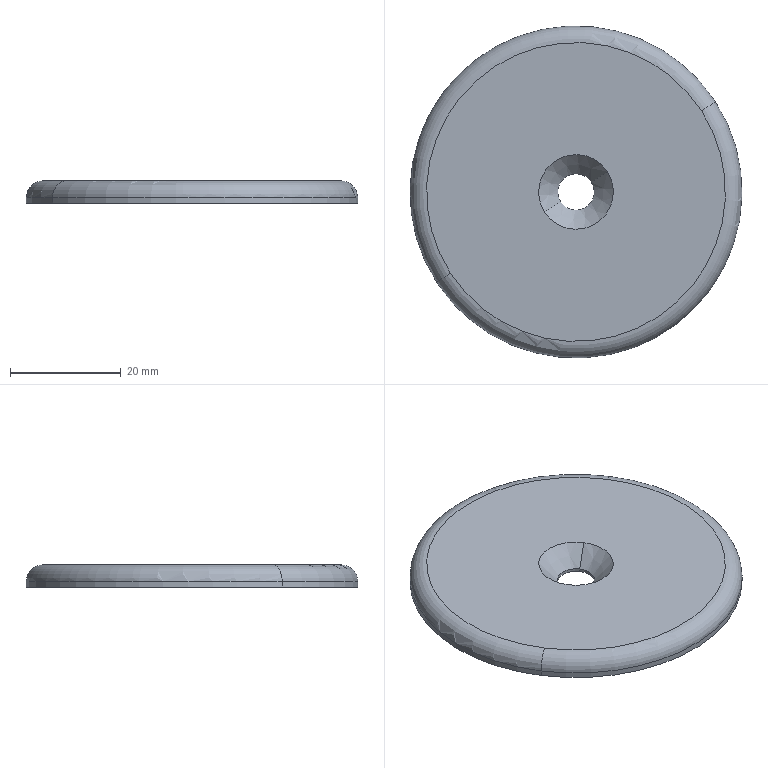Component | SolidWorks | JYTBJ-HeaderPlateAxisBarrelCover-1 | 1 solid | 10 faces | box 60 x 60 x 4 mm | volume 10651 mm3 | cylinder 4 | torus 2 | cone 2 | plane 2 | commonest cylinder face diameters 6.6 x2 60 x2
build123d program:
from build123d import *

# Parameters (mm, degrees)
SKETCH1_R           = 30
BOSS_EXTRUDE1_DEPTH = 2
FILLET1_R           = 3


with BuildPart() as part:
    # Sketch1 → Boss-Extrude1 (new, symmetric)
    with BuildSketch(Plane.XY):
        Circle(SKETCH1_R)
    extrude(amount=BOSS_EXTRUDE1_DEPTH, both=True)

    # Sketch2 → Hole Size according to Hexagon Socket Ra (revolve, cut)
    with BuildSketch(Plane(origin=(0, 0, 2), x_dir=(0, -1, 0), z_dir=(1, 0, 0))):
        Polygon((0, 0), (0, 4), (3.3, 4), (3.3, 3.45), (6.75, 0), align=None)
    revolve(axis=Axis((0, 0, 8.35), (0, 0, -1)), mode=Mode.SUBTRACT)

    # Fillet1
    fillet1_edges = [part.edges().sort_by_distance(p)[0] for p in [
        (-30, 0, 2),
    ]]
    fillet(fillet1_edges, radius=FILLET1_R)


solid = part.part

# Placed as in the assembly
solid = solid.moved(Location((3.373, 96.878, 260.5), (0, 0, 0)))
STEP:
#1=COLOUR_RGB('',0.7922,0.8196,0.9333);
#2=FILL_AREA_STYLE_COLOUR('',#1);
#3=FILL_AREA_STYLE('',(#2));
#4=SURFACE_STYLE_FILL_AREA(#3);
#5=SURFACE_SIDE_STYLE('',(#4));
#6=SURFACE_STYLE_USAGE(.BOTH.,#5);
#7=PRESENTATION_STYLE_ASSIGNMENT((#6));
#8=CARTESIAN_POINT('',(-0.8589,3.173,10.217));
#9=VERTEX_POINT('',#8);
#10=CARTESIAN_POINT('',(1.124,4.456,10.217));
#11=VERTEX_POINT('',#10);
#12=CARTESIAN_POINT('',(0.1328,3.814,10.217));
#13=DIRECTION('',(0.,0.,-1.));
#14=DIRECTION('',(0.8396,0.5432,0.));
#15=AXIS2_PLACEMENT_3D('',#12,#13,#14);
#16=CIRCLE('',#15,1.181);
#17=EDGE_CURVE('',#9,#11,#16,.T.);
#18=ORIENTED_EDGE('',*,*,#17,.F.);
#19=CARTESIAN_POINT('',(-0.7597,3.237,10.335));
#20=VERTEX_POINT('',#19);
#21=CARTESIAN_POINT('',(-0.7597,3.237,10.217));
#22=DIRECTION('',(-0.5432,0.8396,0.));
#23=DIRECTION('',(-0.8396,-0.5432,0.));
#24=AXIS2_PLACEMENT_3D('',#21,#22,#23);
#25=CIRCLE('',#24,0.1181);
#26=EDGE_CURVE('',#9,#20,#25,.T.);
#27=ORIENTED_EDGE('',*,*,#26,.T.);
#28=CARTESIAN_POINT('',(1.025,4.391,10.335));
#29=VERTEX_POINT('',#28);
#30=CARTESIAN_POINT('',(0.1328,3.814,10.335));
#31=DIRECTION('',(0.,0.,1.));
#32=DIRECTION('',(0.8396,0.5432,0.));
#33=AXIS2_PLACEMENT_3D('',#30,#31,#32);
#34=CIRCLE('',#33,1.063);
#35=EDGE_CURVE('',#29,#20,#34,.T.);
#36=ORIENTED_EDGE('',*,*,#35,.F.);
#37=CARTESIAN_POINT('',(1.025,4.391,10.217));
#38=DIRECTION('',(0.5432,-0.8396,0.));
#39=DIRECTION('',(0.8396,0.5432,0.));
#40=AXIS2_PLACEMENT_3D('',#37,#38,#39);
#41=CIRCLE('',#40,0.1181);
#42=EDGE_CURVE('',#11,#29,#41,.T.);
#43=ORIENTED_EDGE('',*,*,#42,.F.);
#44=EDGE_LOOP('',(#18,#27,#36,#43));
#45=FACE_OUTER_BOUND('',#44,.T.);
#46=CARTESIAN_POINT('',(0.1328,3.814,10.217));
#47=DIRECTION('',(0.,0.,1.));
#48=DIRECTION('',(0.8396,0.5432,0.));
#49=AXIS2_PLACEMENT_3D('',#46,#47,#48);
#50=TOROIDAL_SURFACE('',#49,1.063,0.1181);
#51=ADVANCED_FACE('',(#45),#50,.T.);
#52=CARTESIAN_POINT('',(0.02373,3.744,10.199));
#53=VERTEX_POINT('',#52);
#54=CARTESIAN_POINT('',(0.2419,3.885,10.199));
#55=VERTEX_POINT('',#54);
#56=CARTESIAN_POINT('',(0.1328,3.814,10.199));
#57=DIRECTION('',(0.,0.,1.));
#58=DIRECTION('',(0.8396,0.5432,0.));
#59=AXIS2_PLACEMENT_3D('',#56,#57,#58);
#60=CIRCLE('',#59,0.1299);
#61=EDGE_CURVE('',#53,#55,#60,.T.);
#62=ORIENTED_EDGE('',*,*,#61,.F.);
#63=CARTESIAN_POINT('',(-0.09032,3.67,10.335));
#64=VERTEX_POINT('',#63);
#65=CARTESIAN_POINT('',(-0.09032,3.67,10.335));
#66=DIRECTION('',(-0.5937,-0.3841,0.7071));
#67=VECTOR('',#66,39.37);
#68=LINE('',#65,#67);
#69=EDGE_CURVE('',#53,#64,#68,.T.);
#70=ORIENTED_EDGE('',*,*,#69,.T.);
#71=CARTESIAN_POINT('',(0.3559,3.958,10.335));
#72=VERTEX_POINT('',#71);
#73=CARTESIAN_POINT('',(0.1328,3.814,10.335));
#74=DIRECTION('',(0.,0.,1.));
#75=DIRECTION('',(0.8396,0.5432,0.));
#76=AXIS2_PLACEMENT_3D('',#73,#74,#75);
#77=CIRCLE('',#76,0.2657);
#78=EDGE_CURVE('',#64,#72,#77,.T.);
#79=ORIENTED_EDGE('',*,*,#78,.T.);
#80=CARTESIAN_POINT('',(0.3559,3.958,10.335));
#81=DIRECTION('',(0.5937,0.3841,0.7071));
#82=VECTOR('',#81,39.37);
#83=LINE('',#80,#82);
#84=EDGE_CURVE('',#55,#72,#83,.T.);
#85=ORIENTED_EDGE('',*,*,#84,.F.);
#86=EDGE_LOOP('',(#62,#70,#79,#85));
#87=FACE_OUTER_BOUND('',#86,.T.);
#88=CARTESIAN_POINT('',(0.1328,3.814,10.335));
#89=DIRECTION('',(0.,0.,1.));
#90=DIRECTION('',(0.8396,0.5432,0.));
#91=AXIS2_PLACEMENT_3D('',#88,#89,#90);
#92=CONICAL_SURFACE('',#91,0.2657,0.7854);
#93=ADVANCED_FACE('',(#87),#92,.F.);
#94=CARTESIAN_POINT('',(0.02373,3.744,10.177));
#95=VERTEX_POINT('',#94);
#96=CARTESIAN_POINT('',(0.2419,3.885,10.177));
#97=VERTEX_POINT('',#96);
#98=CARTESIAN_POINT('',(0.1328,3.814,10.177));
#99=DIRECTION('',(0.,0.,1.));
#100=DIRECTION('',(0.8396,0.5432,0.));
#101=AXIS2_PLACEMENT_3D('',#98,#99,#100);
#102=CIRCLE('',#101,0.1299);
#103=EDGE_CURVE('',#95,#97,#102,.T.);
#104=ORIENTED_EDGE('',*,*,#103,.F.);
#105=CARTESIAN_POINT('',(0.02373,3.744,10.335));
#106=DIRECTION('',(0.,0.,1.));
#107=VECTOR('',#106,39.37);
#108=LINE('',#105,#107);
#109=EDGE_CURVE('',#95,#53,#108,.T.);
#110=ORIENTED_EDGE('',*,*,#109,.T.);
#111=ORIENTED_EDGE('',*,*,#61,.T.);
#112=CARTESIAN_POINT('',(0.2419,3.885,10.335));
#113=DIRECTION('',(0.,0.,1.));
#114=VECTOR('',#113,39.37);
#115=LINE('',#112,#114);
#116=EDGE_CURVE('',#97,#55,#115,.T.);
#117=ORIENTED_EDGE('',*,*,#116,.F.);
#118=EDGE_LOOP('',(#104,#110,#111,#117));
#119=FACE_OUTER_BOUND('',#118,.T.);
#120=CARTESIAN_POINT('',(0.1328,3.814,10.335));
#121=DIRECTION('',(0.,0.,1.));
#122=DIRECTION('',(0.8396,0.5432,0.));
#123=AXIS2_PLACEMENT_3D('',#120,#121,#122);
#124=CYLINDRICAL_SURFACE('',#123,0.1299);
#125=ADVANCED_FACE('',(#119),#124,.F.);
#126=ORIENTED_EDGE('',*,*,#17,.T.);
#127=CARTESIAN_POINT('',(1.124,4.456,10.177));
#128=VERTEX_POINT('',#127);
#129=CARTESIAN_POINT('',(1.124,4.456,10.335));
#130=DIRECTION('',(0.,0.,-1.));
#131=VECTOR('',#130,39.37);
#132=LINE('',#129,#131);
#133=EDGE_CURVE('',#11,#128,#132,.T.);
#134=ORIENTED_EDGE('',*,*,#133,.T.);
#135=CARTESIAN_POINT('',(-0.8589,3.173,10.177));
#136=VERTEX_POINT('',#135);
#137=CARTESIAN_POINT('',(0.1328,3.814,10.177));
#138=DIRECTION('',(0.,0.,1.));
#139=DIRECTION('',(0.8396,0.5432,0.));
#140=AXIS2_PLACEMENT_3D('',#137,#138,#139);
#141=CIRCLE('',#140,1.181);
#142=EDGE_CURVE('',#128,#136,#141,.T.);
#143=ORIENTED_EDGE('',*,*,#142,.T.);
#144=CARTESIAN_POINT('',(-0.8589,3.173,10.335));
#145=DIRECTION('',(0.,0.,-1.));
#146=VECTOR('',#145,39.37);
#147=LINE('',#144,#146);
#148=EDGE_CURVE('',#9,#136,#147,.T.);
#149=ORIENTED_EDGE('',*,*,#148,.F.);
#150=EDGE_LOOP('',(#126,#134,#143,#149));
#151=FACE_OUTER_BOUND('',#150,.T.);
#152=CARTESIAN_POINT('',(0.1328,3.814,10.335));
#153=DIRECTION('',(0.,0.,-1.));
#154=DIRECTION('',(-0.8396,-0.5432,0.));
#155=AXIS2_PLACEMENT_3D('',#152,#153,#154);
#156=CYLINDRICAL_SURFACE('',#155,1.181);
#157=ADVANCED_FACE('',(#151),#156,.T.);
#158=ORIENTED_EDGE('',*,*,#133,.F.);
#159=CARTESIAN_POINT('',(0.1328,3.814,10.217));
#160=DIRECTION('',(0.,0.,-1.));
#161=DIRECTION('',(0.8396,0.5432,0.));
#162=AXIS2_PLACEMENT_3D('',#159,#160,#161);
#163=CIRCLE('',#162,1.181);
#164=EDGE_CURVE('',#11,#9,#163,.T.);
#165=ORIENTED_EDGE('',*,*,#164,.T.);
#166=ORIENTED_EDGE('',*,*,#148,.T.);
#167=CARTESIAN_POINT('',(0.1328,3.814,10.177));
#168=DIRECTION('',(0.,0.,1.));
#169=DIRECTION('',(0.8396,0.5432,0.));
#170=AXIS2_PLACEMENT_3D('',#167,#168,#169);
#171=CIRCLE('',#170,1.181);
#172=EDGE_CURVE('',#136,#128,#171,.T.);
#173=ORIENTED_EDGE('',*,*,#172,.T.);
#174=EDGE_LOOP('',(#158,#165,#166,#173));
#175=FACE_OUTER_BOUND('',#174,.T.);
#176=CARTESIAN_POINT('',(0.1328,3.814,10.335));
#177=DIRECTION('',(0.,0.,-1.));
#178=DIRECTION('',(-0.8396,-0.5432,0.));
#179=AXIS2_PLACEMENT_3D('',#176,#177,#178);
#180=CYLINDRICAL_SURFACE('',#179,1.181);
#181=ADVANCED_FACE('',(#175),#180,.T.);
#182=ORIENTED_EDGE('',*,*,#35,.T.);
#183=CARTESIAN_POINT('',(0.1328,3.814,10.335));
#184=DIRECTION('',(0.,0.,1.));
#185=DIRECTION('',(0.8396,0.5432,0.));
#186=AXIS2_PLACEMENT_3D('',#183,#184,#185);
#187=CIRCLE('',#186,1.063);
#188=EDGE_CURVE('',#20,#29,#187,.T.);
#189=ORIENTED_EDGE('',*,*,#188,.T.);
#190=EDGE_LOOP('',(#182,#189));
#191=FACE_OUTER_BOUND('',#190,.T.);
#192=CARTESIAN_POINT('',(0.1328,3.814,10.335));
#193=DIRECTION('',(0.,0.,1.));
#194=DIRECTION('',(0.8396,0.5432,0.));
#195=AXIS2_PLACEMENT_3D('',#192,#193,#194);
#196=CIRCLE('',#195,0.2657);
#197=EDGE_CURVE('',#72,#64,#196,.T.);
#198=ORIENTED_EDGE('',*,*,#197,.F.);
#199=ORIENTED_EDGE('',*,*,#78,.F.);
#200=EDGE_LOOP('',(#198,#199));
#201=FACE_BOUND('',#200,.T.);
#202=CARTESIAN_POINT('',(0.1328,3.814,10.335));
#203=DIRECTION('',(0.,0.,1.));
#204=DIRECTION('',(0.8396,0.5432,0.));
#205=AXIS2_PLACEMENT_3D('',#202,#203,#204);
#206=PLANE('',#205);
#207=ADVANCED_FACE('',(#191,#201),#206,.T.);
#208=CARTESIAN_POINT('',(0.1328,3.814,10.177));
#209=DIRECTION('',(0.,0.,1.));
#210=DIRECTION('',(0.8396,0.5432,0.));
#211=AXIS2_PLACEMENT_3D('',#208,#209,#210);
#212=CIRCLE('',#211,0.1299);
#213=EDGE_CURVE('',#97,#95,#212,.T.);
#214=ORIENTED_EDGE('',*,*,#213,.T.);
#215=ORIENTED_EDGE('',*,*,#103,.T.);
#216=EDGE_LOOP('',(#214,#215));
#217=FACE_BOUND('',#216,.T.);
#218=ORIENTED_EDGE('',*,*,#172,.F.);
#219=ORIENTED_EDGE('',*,*,#142,.F.);
#220=EDGE_LOOP('',(#218,#219));
#221=FACE_OUTER_BOUND('',#220,.T.);
#222=CARTESIAN_POINT('',(0.1328,3.814,10.177));
#223=DIRECTION('',(0.,0.,1.));
#224=DIRECTION('',(0.8396,0.5432,0.));
#225=AXIS2_PLACEMENT_3D('',#222,#223,#224);
#226=PLANE('',#225);
#227=ADVANCED_FACE('',(#217,#221),#226,.F.);
#228=ORIENTED_EDGE('',*,*,#109,.F.);
#229=ORIENTED_EDGE('',*,*,#213,.F.);
#230=ORIENTED_EDGE('',*,*,#116,.T.);
#231=CARTESIAN_POINT('',(0.1328,3.814,10.199));
#232=DIRECTION('',(0.,0.,1.));
#233=DIRECTION('',(0.8396,0.5432,0.));
#234=AXIS2_PLACEMENT_3D('',#231,#232,#233);
#235=CIRCLE('',#234,0.1299);
#236=EDGE_CURVE('',#55,#53,#235,.T.);
#237=ORIENTED_EDGE('',*,*,#236,.T.);
#238=EDGE_LOOP('',(#228,#229,#230,#237));
#239=FACE_OUTER_BOUND('',#238,.T.);
#240=CARTESIAN_POINT('',(0.1328,3.814,10.335));
#241=DIRECTION('',(0.,0.,1.));
#242=DIRECTION('',(0.8396,0.5432,0.));
#243=AXIS2_PLACEMENT_3D('',#240,#241,#242);
#244=CYLINDRICAL_SURFACE('',#243,0.1299);
#245=ADVANCED_FACE('',(#239),#244,.F.);
#246=ORIENTED_EDGE('',*,*,#69,.F.);
#247=ORIENTED_EDGE('',*,*,#236,.F.);
#248=ORIENTED_EDGE('',*,*,#84,.T.);
#249=ORIENTED_EDGE('',*,*,#197,.T.);
#250=EDGE_LOOP('',(#246,#247,#248,#249));
#251=FACE_OUTER_BOUND('',#250,.T.);
#252=CARTESIAN_POINT('',(0.1328,3.814,10.335));
#253=DIRECTION('',(0.,0.,1.));
#254=DIRECTION('',(0.8396,0.5432,0.));
#255=AXIS2_PLACEMENT_3D('',#252,#253,#254);
#256=CONICAL_SURFACE('',#255,0.2657,0.7854);
#257=ADVANCED_FACE('',(#251),#256,.F.);
#258=ORIENTED_EDGE('',*,*,#26,.F.);
#259=ORIENTED_EDGE('',*,*,#164,.F.);
#260=ORIENTED_EDGE('',*,*,#42,.T.);
#261=ORIENTED_EDGE('',*,*,#188,.F.);
#262=EDGE_LOOP('',(#258,#259,#260,#261));
#263=FACE_OUTER_BOUND('',#262,.T.);
#264=CARTESIAN_POINT('',(0.1328,3.814,10.217));
#265=DIRECTION('',(0.,0.,1.));
#266=DIRECTION('',(0.8396,0.5432,0.));
#267=AXIS2_PLACEMENT_3D('',#264,#265,#266);
#268=TOROIDAL_SURFACE('',#267,1.063,0.1181);
#269=ADVANCED_FACE('',(#263),#268,.T.);
#270=CLOSED_SHELL('',(#51,#93,#125,#157,#181,#207,#227,#245,#257,#269));
#271=MANIFOLD_SOLID_BREP('',#270);
#272=STYLED_ITEM('',(#7),#271);
#273=PRESENTATION_LAYER_ASSIGNMENT('','',(#272));
#274=CARTESIAN_POINT('',(0.,0.,0.));
#275=DIRECTION('',(0.,0.,1.));
#276=DIRECTION('',(1.,0.,0.));
#277=AXIS2_PLACEMENT_3D('',#274,#275,#276);
#278=(LENGTH_UNIT()NAMED_UNIT(*)SI_UNIT($,.METRE.));
#279=LENGTH_MEASURE_WITH_UNIT(LENGTH_MEASURE(0.0254),#278);
#280=DIMENSIONAL_EXPONENTS(1.,0.,0.,0.,0.,0.,0.);
#281=(CONVERSION_BASED_UNIT('',#279)LENGTH_UNIT()NAMED_UNIT(#280));
#282=UNCERTAINTY_MEASURE_WITH_UNIT(LENGTH_MEASURE(0.00001),#281,'','');
#283=(NAMED_UNIT(*)PLANE_ANGLE_UNIT()SI_UNIT($,.RADIAN.));
#284=(NAMED_UNIT(*)SI_UNIT($,.STERADIAN.)SOLID_ANGLE_UNIT());
#285=(GEOMETRIC_REPRESENTATION_CONTEXT(3)GLOBAL_UNCERTAINTY_ASSIGNED_CONTEXT((#282))GLOBAL_UNIT_ASSIGNED_CONTEXT((#281,#283,#284))REPRESENTATION_CONTEXT('',''));
#286=ADVANCED_BREP_SHAPE_REPRESENTATION('',(#271,#277),#285);
#287=(LENGTH_UNIT()NAMED_UNIT(*)SI_UNIT($,.METRE.));
#288=LENGTH_MEASURE_WITH_UNIT(LENGTH_MEASURE(0.0254),#287);
#289=DIMENSIONAL_EXPONENTS(1.,0.,0.,0.,0.,0.,0.);
#290=(CONVERSION_BASED_UNIT('',#288)LENGTH_UNIT()NAMED_UNIT(#289));
#291=UNCERTAINTY_MEASURE_WITH_UNIT(LENGTH_MEASURE(0.00001),#290,'','');
#292=(NAMED_UNIT(*)PLANE_ANGLE_UNIT()SI_UNIT($,.RADIAN.));
#293=(NAMED_UNIT(*)SI_UNIT($,.STERADIAN.)SOLID_ANGLE_UNIT());
#294=(GEOMETRIC_REPRESENTATION_CONTEXT(3)GLOBAL_UNCERTAINTY_ASSIGNED_CONTEXT((#291))GLOBAL_UNIT_ASSIGNED_CONTEXT((#290,#292,#293))REPRESENTATION_CONTEXT('',''));
#295=MECHANICAL_DESIGN_GEOMETRIC_PRESENTATION_REPRESENTATION('',(#272),#294);